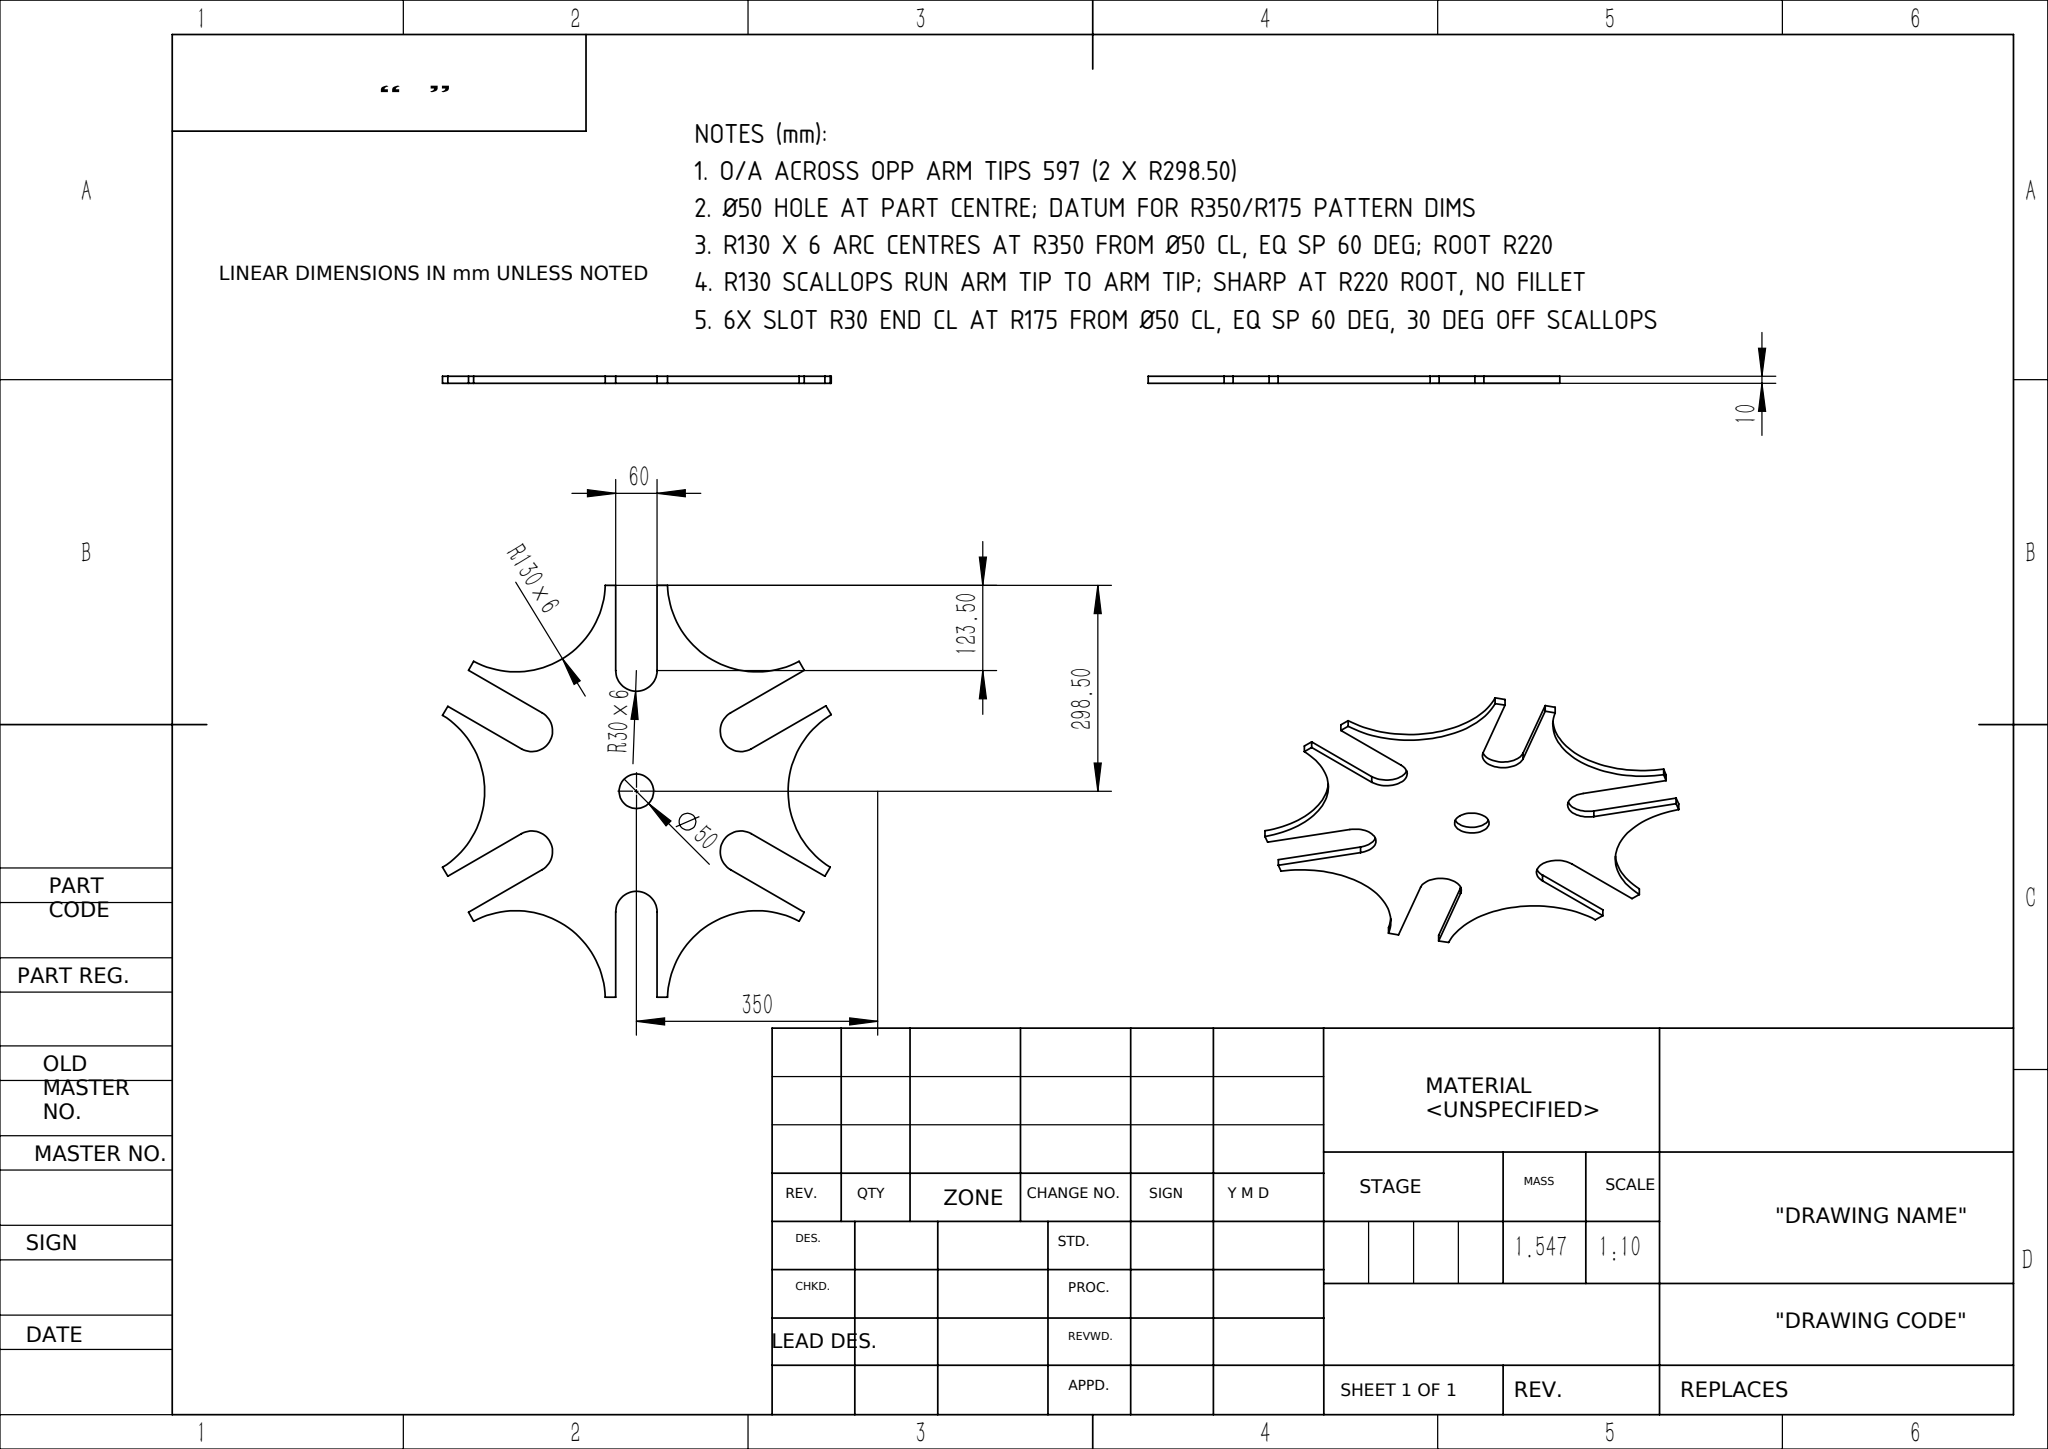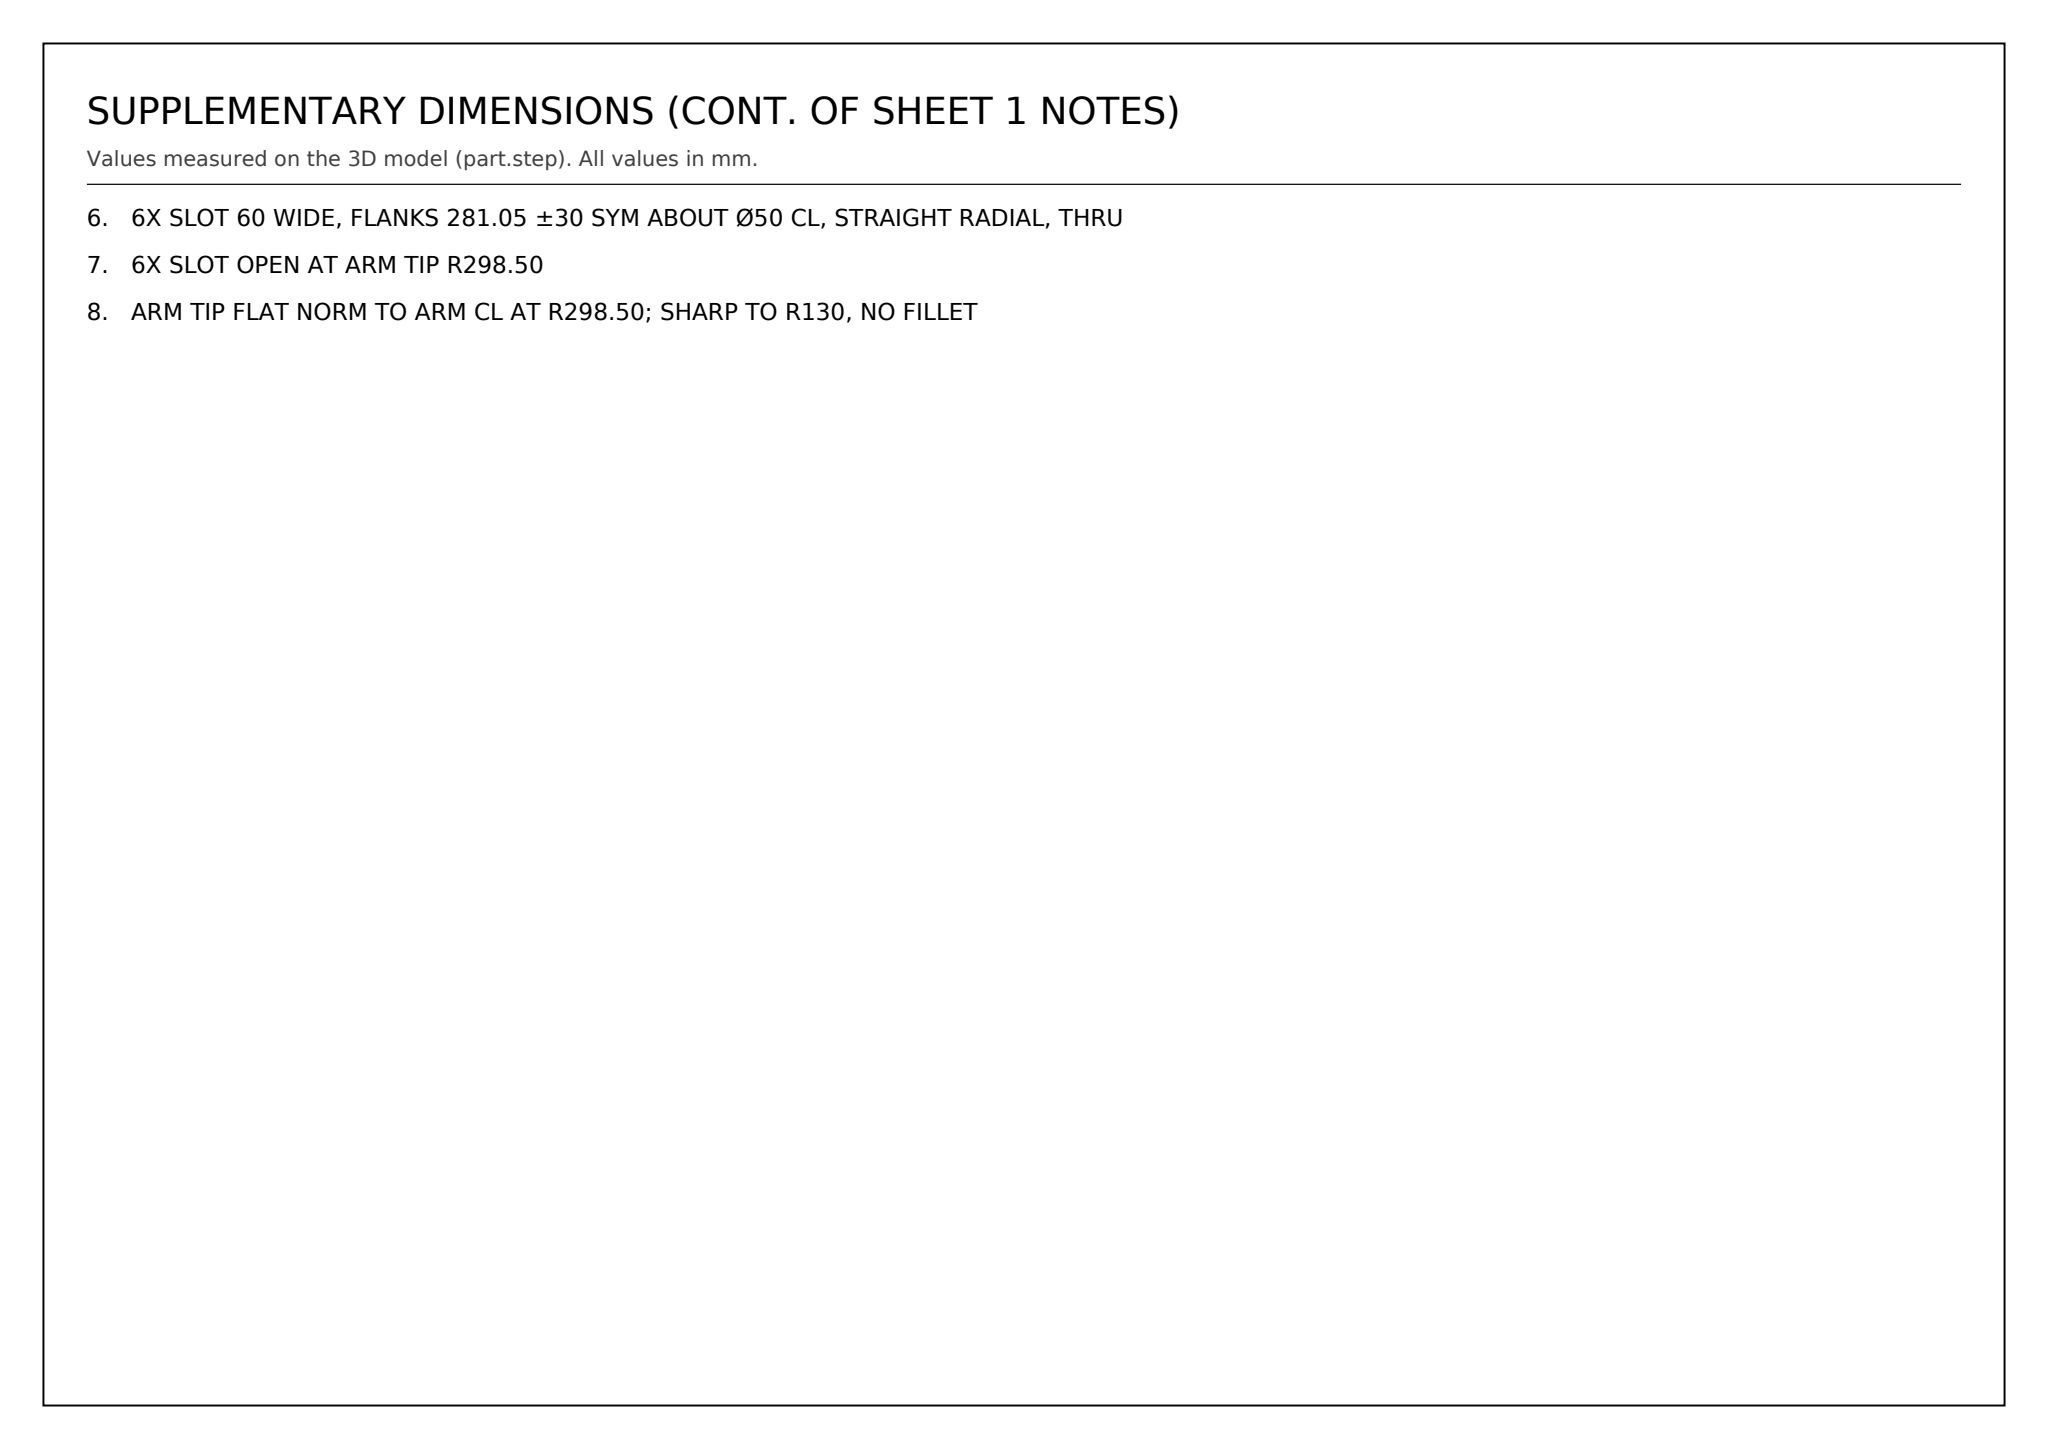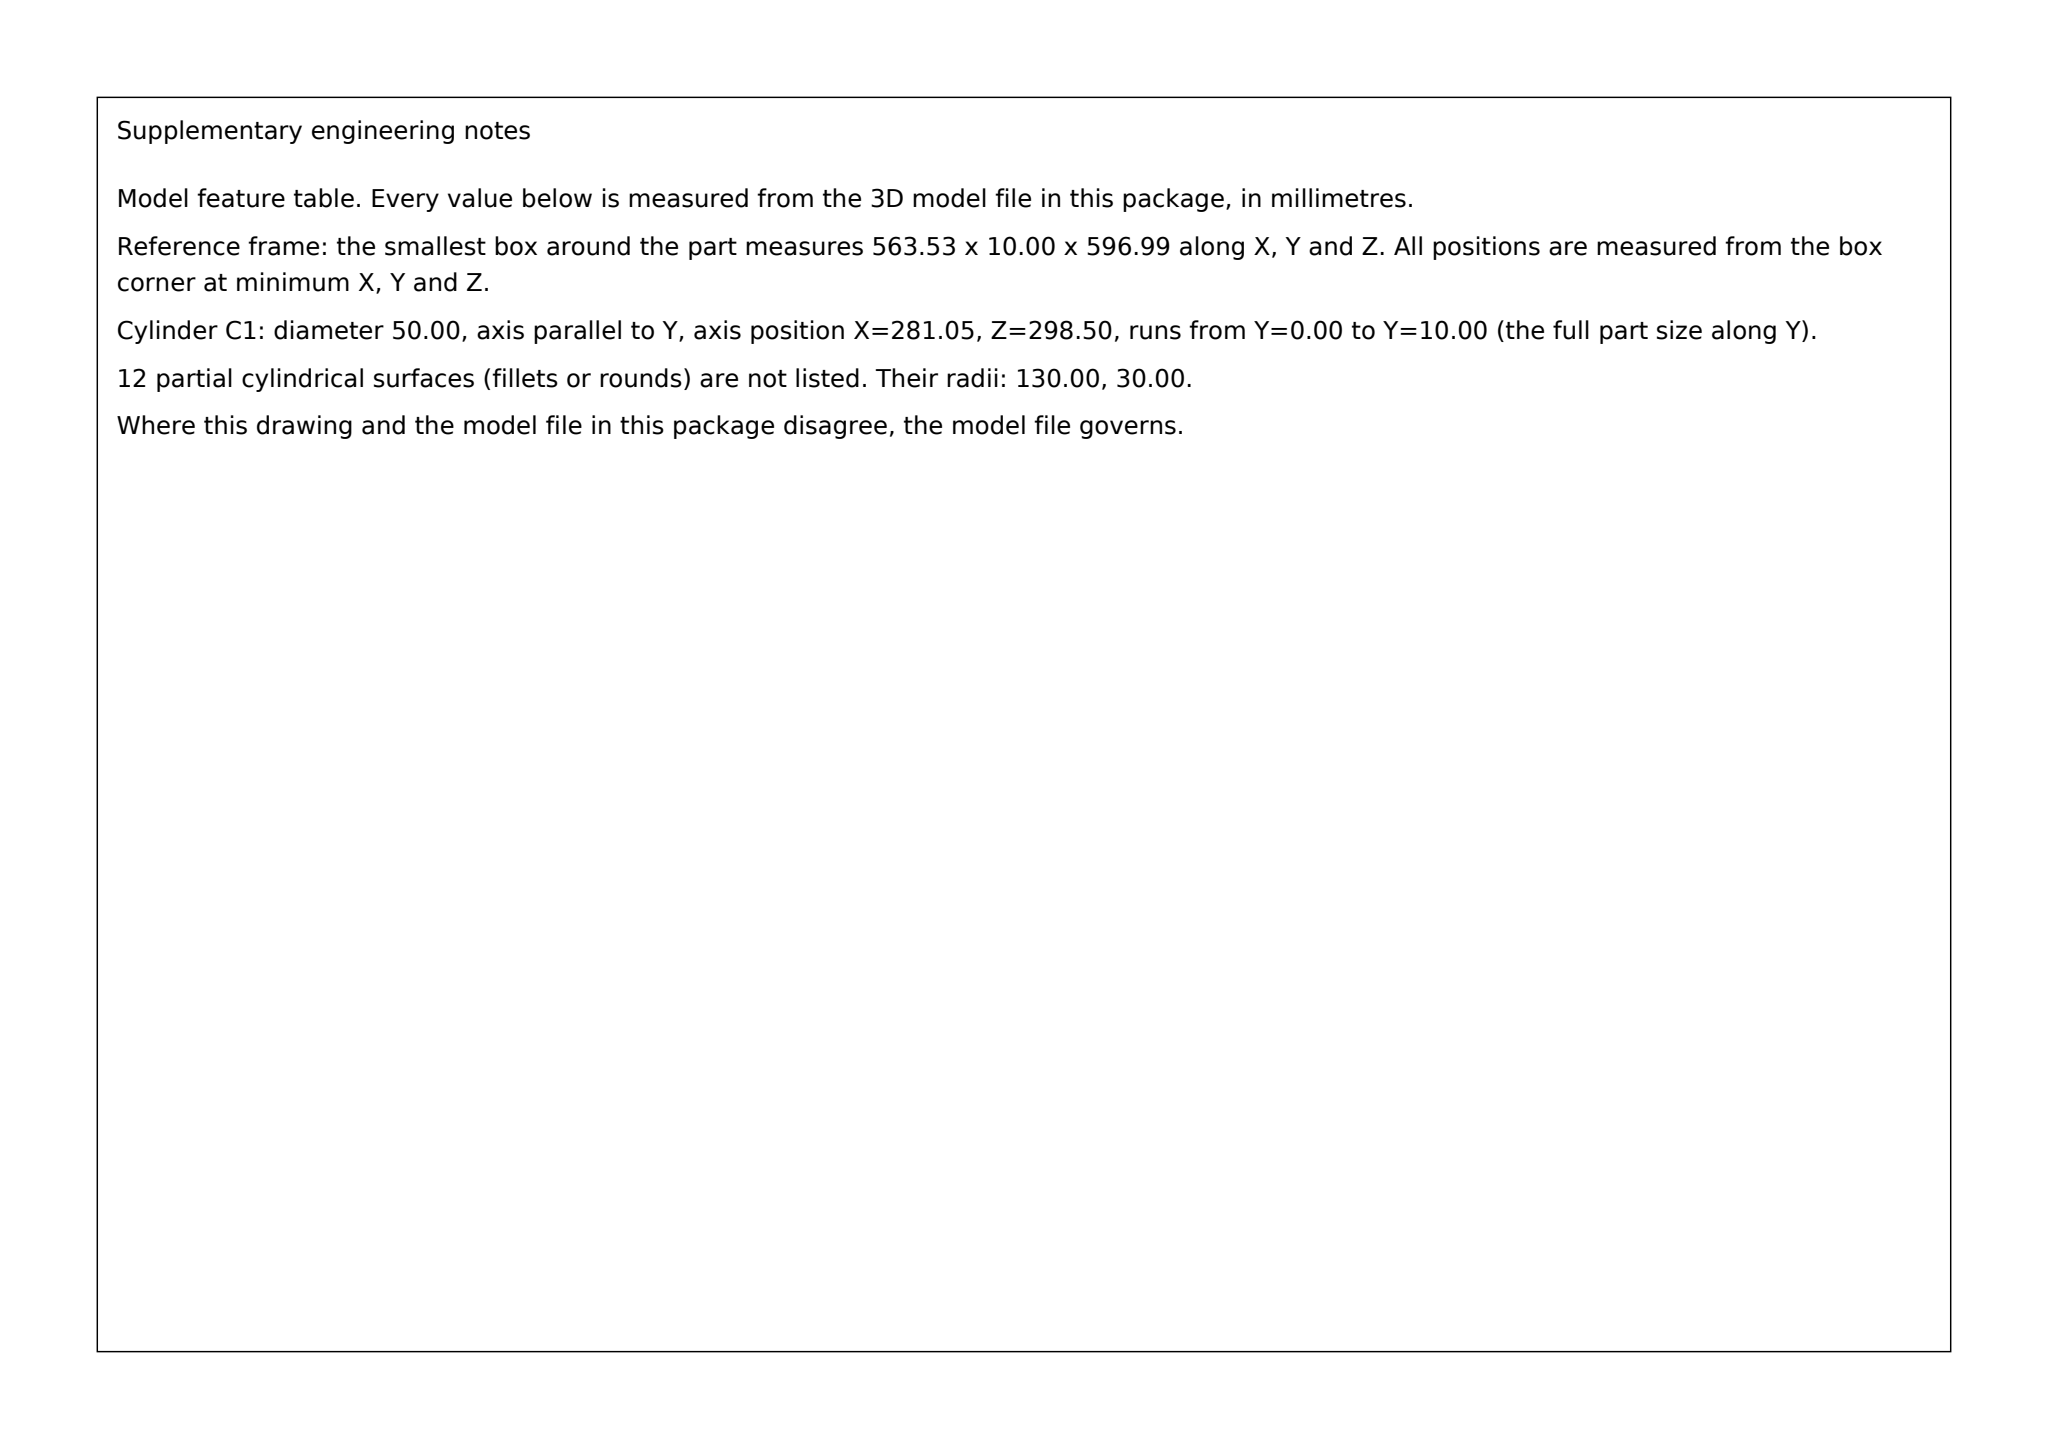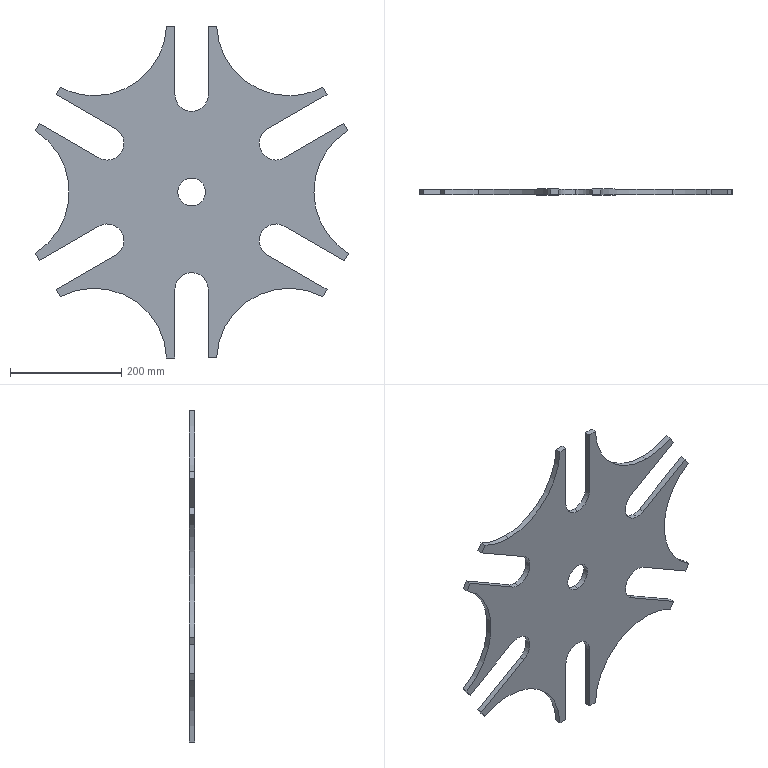Part | SolidWorks | mm | 1 solid | 45 faces | box 563.53 x 10 x 596.99 mm | volume 1547046 mm3 | plane 26 | cylinder 19 | commonest cylinder face diameters 60 x9 260 x8 50 x2
Drawing notes:
O/A ACROSS OPP ARM TIPS 597 (2 X R298.50) | from the solid: bbox_z = 596.992 = 2 x 298.5 tip radius from centre z=298.5
Ø50 HOLE AT PART CENTRE; DATUM FOR R350/R175 PATTERN DIMS | from the solid: Ø50 y-cyl at x=281.05, z=298.5 = symmetry centre of all Ø260/Ø60 patterns
R130 X 6 ARC CENTRES AT R350 FROM Ø50 CL, EQ SP 60 DEG; ROOT R220 | from the solid: Ø260 cyl centres (-68.95,298.5),(106.05,-4.61),(456.05,-4.61),(631.05,298.5),(106.05,601.61),(456.05,601.61) = R350 from (281.05,298.5); 350-130=220
R130 SCALLOPS RUN ARM TIP TO ARM TIP; SHARP AT R220 ROOT, NO FILLET | from the solid: Ø260 cyls meet tip planes z=0/596.99 directly; fillet_radii list empty, no blend faces
6X SLOT R30 END CL AT R175 FROM Ø50 CL, EQ SP 60 DEG, 30 DEG OFF SCALLOPS | from the solid: Ø60 y-cyl centres (281.05,123.5),(281.05,473.5),(129.49,211.0),(129.49,386.0),(432.6,211.0),(432.6,386.0) = R175 from (281.05,298.5)
6X SLOT 60 WIDE, FLANKS 281.05 ±30 SYM ABOUT Ø50 CL, STRAIGHT RADIAL, THRU | from the solid: Planes x=251.05 and x=311.05, 2 faces each, sym about x=281.05; part thickness y=0 to 10; no curved flank faces
6X SLOT OPEN AT ARM TIP R298.50 | from the solid: Slot flank planes x=251.05/311.05 run out to tip planes z=0 and z=596.99
ARM TIP FLAT NORM TO ARM CL AT R298.50; SHARP TO R130, NO FILLET | from the solid: Planes z=0 and z=596.99 (2 faces each, split by slot) at 298.50 from Ø50 CL; fillet_radii empty
build123d program:
from build123d import *

# Parameters (mm, degrees)
SKETCH1_R           = 25
BOSS_EXTRUDE1_DEPTH = 10


with BuildPart() as part:
    # Sketch1 → Boss-Extrude1 (new body)
    with BuildSketch(Plane(origin=(0, 0, 0), x_dir=(1, 0, 0), z_dir=(0, 1, 0))):
        with BuildLine():
            ThreePointArc((106.046, -110.206), (61.281, -62.992), (45, 0))
            ThreePointArc((45, 0), (60.82, 62.152), (104.429, 109.177))
            ThreePointArc((104.429, 109.177), (105.95, 110.146), (107.484, 111.093))
            Line((107.484, 111.093), (99.674, 123.942))
            Line((99.674, 123.942), (98.505, 123.267))
            Line((98.505, 123.267), (-8.446, 61.519))
            ThreePointArc((-8.446, 61.519), (-31.21, 58.522), (-49.426, 72.5))
            ThreePointArc((-49.426, 72.5), (-52.423, 95.265), (-38.446, 113.481))
            Line((-38.446, 113.481), (68.505, 175.229))
            Line((68.505, 175.229), (60.964, 188.29))
            ThreePointArc((60.964, 188.29), (-64.168, 190.049), (-129.836, 296.581))
            ThreePointArc((-129.836, 296.581), (-129.881, 297.538), (-129.918, 298.496))
            Line((-129.918, 298.496), (-145, 298.496))
            Line((-145, 298.496), (-145, 175))
            ThreePointArc((-145, 175), (-153.787, 153.787), (-175, 145))
            ThreePointArc((-175, 145), (-196.213, 153.787), (-205, 175))
            Line((-205, 175), (-205, 298.496))
            Line((-205, 298.496), (-220.082, 298.496))
            ThreePointArc((-220.082, 298.496), (-284.172, 191.008), (-409.265, 187.404))
            ThreePointArc((-409.265, 187.404), (-410.116, 187.844), (-410.964, 188.29))
            Line((-410.964, 188.29), (-418.505, 175.229))
            Line((-418.505, 175.229), (-311.554, 113.481))
            ThreePointArc((-311.554, 113.481), (-297.577, 95.265), (-300.574, 72.5))
            ThreePointArc((-300.574, 72.5), (-318.79, 58.522), (-341.554, 61.519))
            Line((-341.554, 61.519), (-448.505, 123.267))
            Line((-448.505, 123.267), (-456.046, 110.206))
            ThreePointArc((-456.046, 110.206), (-395.004, 0.9586), (-454.429, -109.177))
            ThreePointArc((-454.429, -109.177), (-455.236, -109.695), (-456.046, -110.206))
            Line((-456.046, -110.206), (-448.505, -123.267))
            Line((-448.505, -123.267), (-341.554, -61.519))
            ThreePointArc((-341.554, -61.519), (-318.79, -58.522), (-300.574, -72.5))
            ThreePointArc((-300.574, -72.5), (-297.577, -95.265), (-311.554, -113.481))
            Line((-311.554, -113.481), (-418.505, -175.229))
            Line((-418.505, -175.229), (-410.964, -188.29))
            ThreePointArc((-410.964, -188.29), (-285.832, -190.049), (-220.164, -296.581))
            ThreePointArc((-220.164, -296.581), (-220.119, -297.538), (-220.082, -298.496))
            Line((-220.082, -298.496), (-205, -298.496))
            Line((-205, -298.496), (-205, -175))
            ThreePointArc((-205, -175), (-196.213, -153.787), (-175, -145))
            ThreePointArc((-175, -145), (-153.787, -153.787), (-145, -175))
            Line((-145, -175), (-145, -298.496))
            Line((-145, -298.496), (-129.918, -298.496))
            ThreePointArc((-129.918, -298.496), (-65.828, -191.008), (59.265, -187.404))
            ThreePointArc((59.265, -187.404), (60.116, -187.844), (60.964, -188.29))
            Line((60.964, -188.29), (68.505, -175.229))
            Line((68.505, -175.229), (-38.446, -113.481))
            ThreePointArc((-38.446, -113.481), (-52.423, -95.265), (-49.426, -72.5))
            ThreePointArc((-49.426, -72.5), (-31.21, -58.522), (-8.446, -61.519))
            Line((-8.446, -61.519), (98.505, -123.267))
            Line((98.505, -123.267), (106.046, -110.206))
        make_face()
        with Locations(Location((-175, 0, 0), (0, 0, 270))):
            Circle(SKETCH1_R, mode=Mode.SUBTRACT)
    extrude(amount=BOSS_EXTRUDE1_DEPTH)


solid = part.part